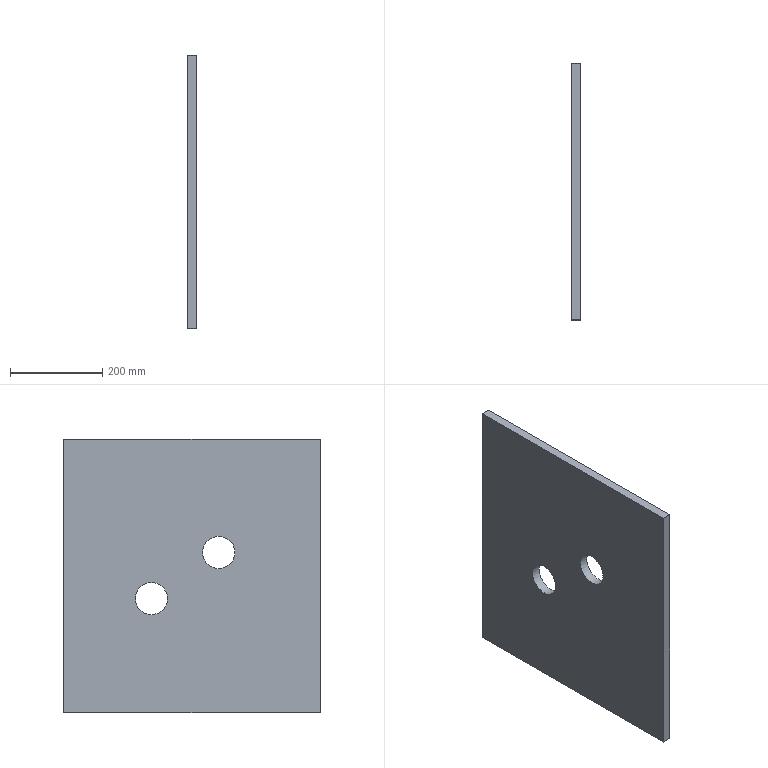Component | NX | BEARING_HOUSING_FIX_PLATE | 1 solid | 8 faces | box 20 x 556 x 594 mm | volume 6451342 mm3 | plane 6 | cylinder 2 | commonest cylinder face diameters 70 x2
STEP:
#1=CARTESIAN_POINT('',(0.,0.,0.));
#2=DIRECTION('',(0.,0.,1.));
#3=DIRECTION('',(1.,0.,0.));
#4=AXIS2_PLACEMENT_3D('',#1,#2,#3);
#5=CARTESIAN_POINT('',(1436.754,3.5,717.5));
#6=VERTEX_POINT('',#5);
#7=CARTESIAN_POINT('',(1436.754,3.5,123.5));
#8=VERTEX_POINT('',#7);
#9=CARTESIAN_POINT('',(1436.754,3.5,717.5));
#10=DIRECTION('',(0.,0.,-1.));
#11=VECTOR('',#10,1.);
#12=LINE('',#9,#11);
#13=CARTESIAN_POINT('',(1456.754,3.5,717.5));
#14=DIRECTION('',(0.,1.,0.));
#15=DIRECTION('',(0.,0.,1.));
#16=AXIS2_PLACEMENT_3D('',#13,#14,#15);
#17=PLANE('',#16);
#18=CARTESIAN_POINT('',(0.,-20.));
#19=DIRECTION('',(-1.,0.));
#20=VECTOR('',#19,1.);
#21=LINE('',#18,#20);
#22=(GEOMETRIC_REPRESENTATION_CONTEXT(2)PARAMETRIC_REPRESENTATION_CONTEXT()REPRESENTATION_CONTEXT('',''));
#23=DEFINITIONAL_REPRESENTATION('',(#21),#22);
#24=PCURVE('',#17,#23);
#25=CARTESIAN_POINT('',(1436.754,223.5,471.5));
#26=DIRECTION('',(1.,0.,0.));
#27=DIRECTION('',(0.,0.,-1.));
#28=AXIS2_PLACEMENT_3D('',#25,#26,#27);
#29=PLANE('',#28);
#30=CARTESIAN_POINT('',(-246.,-220.));
#31=DIRECTION('',(1.,0.));
#32=VECTOR('',#31,1.);
#33=LINE('',#30,#32);
#34=(GEOMETRIC_REPRESENTATION_CONTEXT(2)PARAMETRIC_REPRESENTATION_CONTEXT()REPRESENTATION_CONTEXT('',''));
#35=DEFINITIONAL_REPRESENTATION('',(#33),#34);
#36=PCURVE('',#29,#35);
#37=SURFACE_CURVE('',#12,(#24,#36),.PCURVE_S1.);
#38=EDGE_CURVE('',#6,#8,#37,.T.);
#39=ORIENTED_EDGE('',*,*,#38,.T.);
#40=CARTESIAN_POINT('',(1456.754,3.5,123.5));
#41=VERTEX_POINT('',#40);
#42=CARTESIAN_POINT('',(1456.754,3.5,123.5));
#43=DIRECTION('',(-1.,0.,0.));
#44=VECTOR('',#43,1.);
#45=LINE('',#42,#44);
#46=CARTESIAN_POINT('',(-594.,0.));
#47=DIRECTION('',(0.,-1.));
#48=VECTOR('',#47,1.);
#49=LINE('',#46,#48);
#50=(GEOMETRIC_REPRESENTATION_CONTEXT(2)PARAMETRIC_REPRESENTATION_CONTEXT()REPRESENTATION_CONTEXT('',''));
#51=DEFINITIONAL_REPRESENTATION('',(#49),#50);
#52=PCURVE('',#17,#51);
#53=CARTESIAN_POINT('',(1456.754,3.5,123.5));
#54=DIRECTION('',(0.,0.,1.));
#55=DIRECTION('',(1.,0.,0.));
#56=AXIS2_PLACEMENT_3D('',#53,#54,#55);
#57=PLANE('',#56);
#58=CARTESIAN_POINT('',(0.,0.));
#59=DIRECTION('',(-1.,0.));
#60=VECTOR('',#59,1.);
#61=LINE('',#58,#60);
#62=(GEOMETRIC_REPRESENTATION_CONTEXT(2)PARAMETRIC_REPRESENTATION_CONTEXT()REPRESENTATION_CONTEXT('',''));
#63=DEFINITIONAL_REPRESENTATION('',(#61),#62);
#64=PCURVE('',#57,#63);
#65=SURFACE_CURVE('',#45,(#52,#64),.PCURVE_S1.);
#66=EDGE_CURVE('',#41,#8,#65,.T.);
#67=ORIENTED_EDGE('',*,*,#66,.F.);
#68=CARTESIAN_POINT('',(1456.754,3.5,717.5));
#69=VERTEX_POINT('',#68);
#70=CARTESIAN_POINT('',(1456.754,3.5,717.5));
#71=DIRECTION('',(0.,0.,-1.));
#72=VECTOR('',#71,1.);
#73=LINE('',#70,#72);
#74=CARTESIAN_POINT('',(0.,0.));
#75=DIRECTION('',(-1.,0.));
#76=VECTOR('',#75,1.);
#77=LINE('',#74,#76);
#78=(GEOMETRIC_REPRESENTATION_CONTEXT(2)PARAMETRIC_REPRESENTATION_CONTEXT()REPRESENTATION_CONTEXT('',''));
#79=DEFINITIONAL_REPRESENTATION('',(#77),#78);
#80=PCURVE('',#17,#79);
#81=CARTESIAN_POINT('',(1456.754,223.5,471.5));
#82=DIRECTION('',(1.,0.,0.));
#83=DIRECTION('',(0.,0.,-1.));
#84=AXIS2_PLACEMENT_3D('',#81,#82,#83);
#85=PLANE('',#84);
#86=CARTESIAN_POINT('',(-246.,-220.));
#87=DIRECTION('',(1.,0.));
#88=VECTOR('',#87,1.);
#89=LINE('',#86,#88);
#90=(GEOMETRIC_REPRESENTATION_CONTEXT(2)PARAMETRIC_REPRESENTATION_CONTEXT()REPRESENTATION_CONTEXT('',''));
#91=DEFINITIONAL_REPRESENTATION('',(#89),#90);
#92=PCURVE('',#85,#91);
#93=SURFACE_CURVE('',#73,(#80,#92),.PCURVE_S1.);
#94=EDGE_CURVE('',#69,#41,#93,.T.);
#95=ORIENTED_EDGE('',*,*,#94,.F.);
#96=CARTESIAN_POINT('',(1456.754,3.5,717.5));
#97=DIRECTION('',(-1.,0.,0.));
#98=VECTOR('',#97,1.);
#99=LINE('',#96,#98);
#100=CARTESIAN_POINT('',(0.,0.));
#101=DIRECTION('',(0.,-1.));
#102=VECTOR('',#101,1.);
#103=LINE('',#100,#102);
#104=(GEOMETRIC_REPRESENTATION_CONTEXT(2)PARAMETRIC_REPRESENTATION_CONTEXT()REPRESENTATION_CONTEXT('',''));
#105=DEFINITIONAL_REPRESENTATION('',(#103),#104);
#106=PCURVE('',#17,#105);
#107=CARTESIAN_POINT('',(1456.754,559.5,717.5));
#108=DIRECTION('',(0.,0.,-1.));
#109=DIRECTION('',(-1.,0.,0.));
#110=AXIS2_PLACEMENT_3D('',#107,#108,#109);
#111=PLANE('',#110);
#112=CARTESIAN_POINT('',(0.,-556.));
#113=DIRECTION('',(1.,0.));
#114=VECTOR('',#113,1.);
#115=LINE('',#112,#114);
#116=(GEOMETRIC_REPRESENTATION_CONTEXT(2)PARAMETRIC_REPRESENTATION_CONTEXT()REPRESENTATION_CONTEXT('',''));
#117=DEFINITIONAL_REPRESENTATION('',(#115),#116);
#118=PCURVE('',#111,#117);
#119=SURFACE_CURVE('',#99,(#106,#118),.PCURVE_S1.);
#120=EDGE_CURVE('',#69,#6,#119,.T.);
#121=ORIENTED_EDGE('',*,*,#120,.T.);
#122=EDGE_LOOP('',(#39,#67,#95,#121));
#123=FACE_BOUND('',#122,.T.);
#124=ADVANCED_FACE('',(#123),#17,.F.);
#125=CARTESIAN_POINT('',(1436.754,559.5,123.5));
#126=VERTEX_POINT('',#125);
#127=CARTESIAN_POINT('',(1436.754,3.5,123.5));
#128=DIRECTION('',(0.,1.,0.));
#129=VECTOR('',#128,1.);
#130=LINE('',#127,#129);
#131=CARTESIAN_POINT('',(-20.,0.));
#132=DIRECTION('',(0.,1.));
#133=VECTOR('',#132,1.);
#134=LINE('',#131,#133);
#135=(GEOMETRIC_REPRESENTATION_CONTEXT(2)PARAMETRIC_REPRESENTATION_CONTEXT()REPRESENTATION_CONTEXT('',''));
#136=DEFINITIONAL_REPRESENTATION('',(#134),#135);
#137=PCURVE('',#57,#136);
#138=CARTESIAN_POINT('',(348.,-220.));
#139=DIRECTION('',(0.,1.));
#140=VECTOR('',#139,1.);
#141=LINE('',#138,#140);
#142=(GEOMETRIC_REPRESENTATION_CONTEXT(2)PARAMETRIC_REPRESENTATION_CONTEXT()REPRESENTATION_CONTEXT('',''));
#143=DEFINITIONAL_REPRESENTATION('',(#141),#142);
#144=PCURVE('',#29,#143);
#145=SURFACE_CURVE('',#130,(#137,#144),.PCURVE_S1.);
#146=EDGE_CURVE('',#8,#126,#145,.T.);
#147=ORIENTED_EDGE('',*,*,#146,.T.);
#148=CARTESIAN_POINT('',(1456.754,559.5,123.5));
#149=VERTEX_POINT('',#148);
#150=CARTESIAN_POINT('',(1456.754,559.5,123.5));
#151=DIRECTION('',(-1.,0.,0.));
#152=VECTOR('',#151,1.);
#153=LINE('',#150,#152);
#154=CARTESIAN_POINT('',(0.,556.));
#155=DIRECTION('',(-1.,0.));
#156=VECTOR('',#155,1.);
#157=LINE('',#154,#156);
#158=(GEOMETRIC_REPRESENTATION_CONTEXT(2)PARAMETRIC_REPRESENTATION_CONTEXT()REPRESENTATION_CONTEXT('',''));
#159=DEFINITIONAL_REPRESENTATION('',(#157),#158);
#160=PCURVE('',#57,#159);
#161=CARTESIAN_POINT('',(1456.754,559.5,123.5));
#162=DIRECTION('',(0.,-1.,0.));
#163=DIRECTION('',(0.,0.,-1.));
#164=AXIS2_PLACEMENT_3D('',#161,#162,#163);
#165=PLANE('',#164);
#166=CARTESIAN_POINT('',(0.,0.));
#167=DIRECTION('',(0.,-1.));
#168=VECTOR('',#167,1.);
#169=LINE('',#166,#168);
#170=(GEOMETRIC_REPRESENTATION_CONTEXT(2)PARAMETRIC_REPRESENTATION_CONTEXT()REPRESENTATION_CONTEXT('',''));
#171=DEFINITIONAL_REPRESENTATION('',(#169),#170);
#172=PCURVE('',#165,#171);
#173=SURFACE_CURVE('',#153,(#160,#172),.PCURVE_S1.);
#174=EDGE_CURVE('',#149,#126,#173,.T.);
#175=ORIENTED_EDGE('',*,*,#174,.F.);
#176=CARTESIAN_POINT('',(1456.754,3.5,123.5));
#177=DIRECTION('',(0.,1.,0.));
#178=VECTOR('',#177,1.);
#179=LINE('',#176,#178);
#180=CARTESIAN_POINT('',(0.,0.));
#181=DIRECTION('',(0.,1.));
#182=VECTOR('',#181,1.);
#183=LINE('',#180,#182);
#184=(GEOMETRIC_REPRESENTATION_CONTEXT(2)PARAMETRIC_REPRESENTATION_CONTEXT()REPRESENTATION_CONTEXT('',''));
#185=DEFINITIONAL_REPRESENTATION('',(#183),#184);
#186=PCURVE('',#57,#185);
#187=CARTESIAN_POINT('',(348.,-220.));
#188=DIRECTION('',(0.,1.));
#189=VECTOR('',#188,1.);
#190=LINE('',#187,#189);
#191=(GEOMETRIC_REPRESENTATION_CONTEXT(2)PARAMETRIC_REPRESENTATION_CONTEXT()REPRESENTATION_CONTEXT('',''));
#192=DEFINITIONAL_REPRESENTATION('',(#190),#191);
#193=PCURVE('',#85,#192);
#194=SURFACE_CURVE('',#179,(#186,#193),.PCURVE_S1.);
#195=EDGE_CURVE('',#41,#149,#194,.T.);
#196=ORIENTED_EDGE('',*,*,#195,.F.);
#197=ORIENTED_EDGE('',*,*,#66,.T.);
#198=EDGE_LOOP('',(#147,#175,#196,#197));
#199=FACE_BOUND('',#198,.T.);
#200=ADVANCED_FACE('',(#199),#57,.F.);
#201=CARTESIAN_POINT('',(1436.754,559.5,717.5));
#202=VERTEX_POINT('',#201);
#203=CARTESIAN_POINT('',(1436.754,559.5,123.5));
#204=DIRECTION('',(0.,0.,1.));
#205=VECTOR('',#204,1.);
#206=LINE('',#203,#205);
#207=CARTESIAN_POINT('',(0.,-20.));
#208=DIRECTION('',(-1.,0.));
#209=VECTOR('',#208,1.);
#210=LINE('',#207,#209);
#211=(GEOMETRIC_REPRESENTATION_CONTEXT(2)PARAMETRIC_REPRESENTATION_CONTEXT()REPRESENTATION_CONTEXT('',''));
#212=DEFINITIONAL_REPRESENTATION('',(#210),#211);
#213=PCURVE('',#165,#212);
#214=CARTESIAN_POINT('',(348.,336.));
#215=DIRECTION('',(-1.,0.));
#216=VECTOR('',#215,1.);
#217=LINE('',#214,#216);
#218=(GEOMETRIC_REPRESENTATION_CONTEXT(2)PARAMETRIC_REPRESENTATION_CONTEXT()REPRESENTATION_CONTEXT('',''));
#219=DEFINITIONAL_REPRESENTATION('',(#217),#218);
#220=PCURVE('',#29,#219);
#221=SURFACE_CURVE('',#206,(#213,#220),.PCURVE_S1.);
#222=EDGE_CURVE('',#126,#202,#221,.T.);
#223=ORIENTED_EDGE('',*,*,#222,.T.);
#224=CARTESIAN_POINT('',(1456.754,559.5,717.5));
#225=VERTEX_POINT('',#224);
#226=CARTESIAN_POINT('',(1456.754,559.5,717.5));
#227=DIRECTION('',(-1.,0.,0.));
#228=VECTOR('',#227,1.);
#229=LINE('',#226,#228);
#230=CARTESIAN_POINT('',(-594.,0.));
#231=DIRECTION('',(0.,-1.));
#232=VECTOR('',#231,1.);
#233=LINE('',#230,#232);
#234=(GEOMETRIC_REPRESENTATION_CONTEXT(2)PARAMETRIC_REPRESENTATION_CONTEXT()REPRESENTATION_CONTEXT('',''));
#235=DEFINITIONAL_REPRESENTATION('',(#233),#234);
#236=PCURVE('',#165,#235);
#237=CARTESIAN_POINT('',(0.,0.));
#238=DIRECTION('',(1.,0.));
#239=VECTOR('',#238,1.);
#240=LINE('',#237,#239);
#241=(GEOMETRIC_REPRESENTATION_CONTEXT(2)PARAMETRIC_REPRESENTATION_CONTEXT()REPRESENTATION_CONTEXT('',''));
#242=DEFINITIONAL_REPRESENTATION('',(#240),#241);
#243=PCURVE('',#111,#242);
#244=SURFACE_CURVE('',#229,(#236,#243),.PCURVE_S1.);
#245=EDGE_CURVE('',#225,#202,#244,.T.);
#246=ORIENTED_EDGE('',*,*,#245,.F.);
#247=CARTESIAN_POINT('',(1456.754,559.5,123.5));
#248=DIRECTION('',(0.,0.,1.));
#249=VECTOR('',#248,1.);
#250=LINE('',#247,#249);
#251=CARTESIAN_POINT('',(0.,0.));
#252=DIRECTION('',(-1.,0.));
#253=VECTOR('',#252,1.);
#254=LINE('',#251,#253);
#255=(GEOMETRIC_REPRESENTATION_CONTEXT(2)PARAMETRIC_REPRESENTATION_CONTEXT()REPRESENTATION_CONTEXT('',''));
#256=DEFINITIONAL_REPRESENTATION('',(#254),#255);
#257=PCURVE('',#165,#256);
#258=CARTESIAN_POINT('',(348.,336.));
#259=DIRECTION('',(-1.,0.));
#260=VECTOR('',#259,1.);
#261=LINE('',#258,#260);
#262=(GEOMETRIC_REPRESENTATION_CONTEXT(2)PARAMETRIC_REPRESENTATION_CONTEXT()REPRESENTATION_CONTEXT('',''));
#263=DEFINITIONAL_REPRESENTATION('',(#261),#262);
#264=PCURVE('',#85,#263);
#265=SURFACE_CURVE('',#250,(#257,#264),.PCURVE_S1.);
#266=EDGE_CURVE('',#149,#225,#265,.T.);
#267=ORIENTED_EDGE('',*,*,#266,.F.);
#268=ORIENTED_EDGE('',*,*,#174,.T.);
#269=EDGE_LOOP('',(#223,#246,#267,#268));
#270=FACE_BOUND('',#269,.T.);
#271=ADVANCED_FACE('',(#270),#165,.F.);
#272=CARTESIAN_POINT('',(1456.754,258.5,471.5));
#273=VERTEX_POINT('',#272);
#274=CARTESIAN_POINT('',(1456.754,223.5,471.5));
#275=DIRECTION('',(1.,0.,0.));
#276=DIRECTION('',(0.,1.,0.));
#277=AXIS2_PLACEMENT_3D('',#274,#275,#276);
#278=CIRCLE('',#277,35.);
#279=CARTESIAN_POINT('',(1456.754,223.5,471.5));
#280=DIRECTION('',(-1.,0.,0.));
#281=DIRECTION('',(0.,0.,1.));
#282=AXIS2_PLACEMENT_3D('',#279,#280,#281);
#283=CYLINDRICAL_SURFACE('',#282,35.);
#284=CARTESIAN_POINT('',(7.854,0.));
#285=DIRECTION('',(-1.,0.));
#286=VECTOR('',#285,1.);
#287=LINE('',#284,#286);
#288=(GEOMETRIC_REPRESENTATION_CONTEXT(2)PARAMETRIC_REPRESENTATION_CONTEXT()REPRESENTATION_CONTEXT('',''));
#289=DEFINITIONAL_REPRESENTATION('',(#287),#288);
#290=PCURVE('',#283,#289);
#291=CARTESIAN_POINT('',(0.,0.));
#292=DIRECTION('',(0.,1.));
#293=AXIS2_PLACEMENT_2D('',#291,#292);
#294=CIRCLE('',#293,35.);
#295=(GEOMETRIC_REPRESENTATION_CONTEXT(2)PARAMETRIC_REPRESENTATION_CONTEXT()REPRESENTATION_CONTEXT('',''));
#296=DEFINITIONAL_REPRESENTATION('',(#294),#295);
#297=PCURVE('',#85,#296);
#298=SURFACE_CURVE('',#278,(#290,#297),.PCURVE_S1.);
#299=EDGE_CURVE('',#273,#273,#298,.T.);
#300=ORIENTED_EDGE('',*,*,#299,.F.);
#301=CARTESIAN_POINT('',(1436.754,258.5,471.5));
#302=VERTEX_POINT('',#301);
#303=CARTESIAN_POINT('',(1456.754,258.5,471.5));
#304=CARTESIAN_POINT('',(1436.754,258.5,471.5));
#305=B_SPLINE_CURVE_WITH_KNOTS('',1,(#303,#304),.UNSPECIFIED.,.F.,.F.,(2,2),(0.,20.),.PIECEWISE_BEZIER_KNOTS.);
#306=CARTESIAN_POINT('',(7.854,0.));
#307=DIRECTION('',(0.,1.));
#308=VECTOR('',#307,1.);
#309=LINE('',#306,#308);
#310=(GEOMETRIC_REPRESENTATION_CONTEXT(2)PARAMETRIC_REPRESENTATION_CONTEXT()REPRESENTATION_CONTEXT('',''));
#311=DEFINITIONAL_REPRESENTATION('',(#309),#310);
#312=PCURVE('',#283,#311);
#313=CARTESIAN_POINT('',(1.571,0.));
#314=DIRECTION('',(0.,1.));
#315=VECTOR('',#314,1.);
#316=LINE('',#313,#315);
#317=(GEOMETRIC_REPRESENTATION_CONTEXT(2)PARAMETRIC_REPRESENTATION_CONTEXT()REPRESENTATION_CONTEXT('',''));
#318=DEFINITIONAL_REPRESENTATION('',(#316),#317);
#319=PCURVE('',#283,#318);
#320=SEAM_CURVE('',#305,(#312,#319),.PCURVE_S1.);
#321=EDGE_CURVE('',#273,#302,#320,.T.);
#322=ORIENTED_EDGE('',*,*,#321,.T.);
#323=CARTESIAN_POINT('',(1436.754,223.5,471.5));
#324=DIRECTION('',(1.,0.,0.));
#325=DIRECTION('',(0.,1.,0.));
#326=AXIS2_PLACEMENT_3D('',#323,#324,#325);
#327=CIRCLE('',#326,35.);
#328=CARTESIAN_POINT('',(7.854,20.));
#329=DIRECTION('',(-1.,0.));
#330=VECTOR('',#329,1.);
#331=LINE('',#328,#330);
#332=(GEOMETRIC_REPRESENTATION_CONTEXT(2)PARAMETRIC_REPRESENTATION_CONTEXT()REPRESENTATION_CONTEXT('',''));
#333=DEFINITIONAL_REPRESENTATION('',(#331),#332);
#334=PCURVE('',#283,#333);
#335=CARTESIAN_POINT('',(0.,0.));
#336=DIRECTION('',(0.,1.));
#337=AXIS2_PLACEMENT_2D('',#335,#336);
#338=CIRCLE('',#337,35.);
#339=(GEOMETRIC_REPRESENTATION_CONTEXT(2)PARAMETRIC_REPRESENTATION_CONTEXT()REPRESENTATION_CONTEXT('',''));
#340=DEFINITIONAL_REPRESENTATION('',(#338),#339);
#341=PCURVE('',#29,#340);
#342=SURFACE_CURVE('',#327,(#334,#341),.PCURVE_S1.);
#343=EDGE_CURVE('',#302,#302,#342,.T.);
#344=ORIENTED_EDGE('',*,*,#343,.T.);
#345=ORIENTED_EDGE('',*,*,#321,.F.);
#346=EDGE_LOOP('',(#300,#322,#344,#345));
#347=FACE_BOUND('',#346,.F.);
#348=ADVANCED_FACE('',(#347),#283,.F.);
#349=CARTESIAN_POINT('',(1436.754,559.5,717.5));
#350=DIRECTION('',(0.,-1.,0.));
#351=VECTOR('',#350,1.);
#352=LINE('',#349,#351);
#353=CARTESIAN_POINT('',(20.,0.));
#354=DIRECTION('',(0.,-1.));
#355=VECTOR('',#354,1.);
#356=LINE('',#353,#355);
#357=(GEOMETRIC_REPRESENTATION_CONTEXT(2)PARAMETRIC_REPRESENTATION_CONTEXT()REPRESENTATION_CONTEXT('',''));
#358=DEFINITIONAL_REPRESENTATION('',(#356),#357);
#359=PCURVE('',#111,#358);
#360=CARTESIAN_POINT('',(-246.,336.));
#361=DIRECTION('',(0.,-1.));
#362=VECTOR('',#361,1.);
#363=LINE('',#360,#362);
#364=(GEOMETRIC_REPRESENTATION_CONTEXT(2)PARAMETRIC_REPRESENTATION_CONTEXT()REPRESENTATION_CONTEXT('',''));
#365=DEFINITIONAL_REPRESENTATION('',(#363),#364);
#366=PCURVE('',#29,#365);
#367=SURFACE_CURVE('',#352,(#359,#366),.PCURVE_S1.);
#368=EDGE_CURVE('',#202,#6,#367,.T.);
#369=ORIENTED_EDGE('',*,*,#368,.T.);
#370=ORIENTED_EDGE('',*,*,#120,.F.);
#371=CARTESIAN_POINT('',(1456.754,559.5,717.5));
#372=DIRECTION('',(0.,-1.,0.));
#373=VECTOR('',#372,1.);
#374=LINE('',#371,#373);
#375=CARTESIAN_POINT('',(0.,0.));
#376=DIRECTION('',(0.,-1.));
#377=VECTOR('',#376,1.);
#378=LINE('',#375,#377);
#379=(GEOMETRIC_REPRESENTATION_CONTEXT(2)PARAMETRIC_REPRESENTATION_CONTEXT()REPRESENTATION_CONTEXT('',''));
#380=DEFINITIONAL_REPRESENTATION('',(#378),#379);
#381=PCURVE('',#111,#380);
#382=CARTESIAN_POINT('',(-246.,336.));
#383=DIRECTION('',(0.,-1.));
#384=VECTOR('',#383,1.);
#385=LINE('',#382,#384);
#386=(GEOMETRIC_REPRESENTATION_CONTEXT(2)PARAMETRIC_REPRESENTATION_CONTEXT()REPRESENTATION_CONTEXT('',''));
#387=DEFINITIONAL_REPRESENTATION('',(#385),#386);
#388=PCURVE('',#85,#387);
#389=SURFACE_CURVE('',#374,(#381,#388),.PCURVE_S1.);
#390=EDGE_CURVE('',#225,#69,#389,.T.);
#391=ORIENTED_EDGE('',*,*,#390,.F.);
#392=ORIENTED_EDGE('',*,*,#245,.T.);
#393=EDGE_LOOP('',(#369,#370,#391,#392));
#394=FACE_BOUND('',#393,.T.);
#395=ADVANCED_FACE('',(#394),#111,.F.);
#396=CARTESIAN_POINT('',(1456.754,404.5,371.5));
#397=VERTEX_POINT('',#396);
#398=CARTESIAN_POINT('',(1456.754,369.5,371.5));
#399=DIRECTION('',(1.,0.,0.));
#400=DIRECTION('',(0.,1.,0.));
#401=AXIS2_PLACEMENT_3D('',#398,#399,#400);
#402=CIRCLE('',#401,35.);
#403=CARTESIAN_POINT('',(1456.754,369.5,371.5));
#404=DIRECTION('',(-1.,0.,0.));
#405=DIRECTION('',(0.,0.,1.));
#406=AXIS2_PLACEMENT_3D('',#403,#404,#405);
#407=CYLINDRICAL_SURFACE('',#406,35.);
#408=CARTESIAN_POINT('',(7.854,0.));
#409=DIRECTION('',(-1.,0.));
#410=VECTOR('',#409,1.);
#411=LINE('',#408,#410);
#412=(GEOMETRIC_REPRESENTATION_CONTEXT(2)PARAMETRIC_REPRESENTATION_CONTEXT()REPRESENTATION_CONTEXT('',''));
#413=DEFINITIONAL_REPRESENTATION('',(#411),#412);
#414=PCURVE('',#407,#413);
#415=CARTESIAN_POINT('',(100.,146.));
#416=DIRECTION('',(0.,1.));
#417=AXIS2_PLACEMENT_2D('',#415,#416);
#418=CIRCLE('',#417,35.);
#419=(GEOMETRIC_REPRESENTATION_CONTEXT(2)PARAMETRIC_REPRESENTATION_CONTEXT()REPRESENTATION_CONTEXT('',''));
#420=DEFINITIONAL_REPRESENTATION('',(#418),#419);
#421=PCURVE('',#85,#420);
#422=SURFACE_CURVE('',#402,(#414,#421),.PCURVE_S1.);
#423=EDGE_CURVE('',#397,#397,#422,.T.);
#424=ORIENTED_EDGE('',*,*,#423,.F.);
#425=CARTESIAN_POINT('',(1436.754,404.5,371.5));
#426=VERTEX_POINT('',#425);
#427=CARTESIAN_POINT('',(1456.754,404.5,371.5));
#428=CARTESIAN_POINT('',(1436.754,404.5,371.5));
#429=B_SPLINE_CURVE_WITH_KNOTS('',1,(#427,#428),.UNSPECIFIED.,.F.,.F.,(2,2),(0.,20.),.PIECEWISE_BEZIER_KNOTS.);
#430=CARTESIAN_POINT('',(7.854,0.));
#431=DIRECTION('',(0.,1.));
#432=VECTOR('',#431,1.);
#433=LINE('',#430,#432);
#434=(GEOMETRIC_REPRESENTATION_CONTEXT(2)PARAMETRIC_REPRESENTATION_CONTEXT()REPRESENTATION_CONTEXT('',''));
#435=DEFINITIONAL_REPRESENTATION('',(#433),#434);
#436=PCURVE('',#407,#435);
#437=CARTESIAN_POINT('',(1.571,0.));
#438=DIRECTION('',(0.,1.));
#439=VECTOR('',#438,1.);
#440=LINE('',#437,#439);
#441=(GEOMETRIC_REPRESENTATION_CONTEXT(2)PARAMETRIC_REPRESENTATION_CONTEXT()REPRESENTATION_CONTEXT('',''));
#442=DEFINITIONAL_REPRESENTATION('',(#440),#441);
#443=PCURVE('',#407,#442);
#444=SEAM_CURVE('',#429,(#436,#443),.PCURVE_S1.);
#445=EDGE_CURVE('',#397,#426,#444,.T.);
#446=ORIENTED_EDGE('',*,*,#445,.T.);
#447=CARTESIAN_POINT('',(1436.754,369.5,371.5));
#448=DIRECTION('',(1.,0.,0.));
#449=DIRECTION('',(0.,1.,0.));
#450=AXIS2_PLACEMENT_3D('',#447,#448,#449);
#451=CIRCLE('',#450,35.);
#452=CARTESIAN_POINT('',(7.854,20.));
#453=DIRECTION('',(-1.,0.));
#454=VECTOR('',#453,1.);
#455=LINE('',#452,#454);
#456=(GEOMETRIC_REPRESENTATION_CONTEXT(2)PARAMETRIC_REPRESENTATION_CONTEXT()REPRESENTATION_CONTEXT('',''));
#457=DEFINITIONAL_REPRESENTATION('',(#455),#456);
#458=PCURVE('',#407,#457);
#459=CARTESIAN_POINT('',(100.,146.));
#460=DIRECTION('',(0.,1.));
#461=AXIS2_PLACEMENT_2D('',#459,#460);
#462=CIRCLE('',#461,35.);
#463=(GEOMETRIC_REPRESENTATION_CONTEXT(2)PARAMETRIC_REPRESENTATION_CONTEXT()REPRESENTATION_CONTEXT('',''));
#464=DEFINITIONAL_REPRESENTATION('',(#462),#463);
#465=PCURVE('',#29,#464);
#466=SURFACE_CURVE('',#451,(#458,#465),.PCURVE_S1.);
#467=EDGE_CURVE('',#426,#426,#466,.T.);
#468=ORIENTED_EDGE('',*,*,#467,.T.);
#469=ORIENTED_EDGE('',*,*,#445,.F.);
#470=EDGE_LOOP('',(#424,#446,#468,#469));
#471=FACE_BOUND('',#470,.F.);
#472=ADVANCED_FACE('',(#471),#407,.F.);
#473=ORIENTED_EDGE('',*,*,#94,.T.);
#474=ORIENTED_EDGE('',*,*,#195,.T.);
#475=ORIENTED_EDGE('',*,*,#266,.T.);
#476=ORIENTED_EDGE('',*,*,#390,.T.);
#477=EDGE_LOOP('',(#473,#474,#475,#476));
#478=FACE_BOUND('',#477,.T.);
#479=ORIENTED_EDGE('',*,*,#299,.F.);
#480=EDGE_LOOP('',(#479));
#481=FACE_BOUND('',#480,.T.);
#482=ORIENTED_EDGE('',*,*,#423,.F.);
#483=EDGE_LOOP('',(#482));
#484=FACE_BOUND('',#483,.T.);
#485=ADVANCED_FACE('',(#478,#481,#484),#85,.T.);
#486=ORIENTED_EDGE('',*,*,#38,.F.);
#487=ORIENTED_EDGE('',*,*,#368,.F.);
#488=ORIENTED_EDGE('',*,*,#222,.F.);
#489=ORIENTED_EDGE('',*,*,#146,.F.);
#490=EDGE_LOOP('',(#486,#487,#488,#489));
#491=FACE_BOUND('',#490,.T.);
#492=ORIENTED_EDGE('',*,*,#343,.T.);
#493=EDGE_LOOP('',(#492));
#494=FACE_BOUND('',#493,.T.);
#495=ORIENTED_EDGE('',*,*,#467,.T.);
#496=EDGE_LOOP('',(#495));
#497=FACE_BOUND('',#496,.T.);
#498=ADVANCED_FACE('',(#491,#494,#497),#29,.F.);
#499=CLOSED_SHELL('',(#124,#200,#271,#348,#395,#472,#485,#498));
#500=MANIFOLD_SOLID_BREP('',#499);
#501=(LENGTH_UNIT()NAMED_UNIT(*)SI_UNIT(.MILLI.,.METRE.));
#502=UNCERTAINTY_MEASURE_WITH_UNIT(LENGTH_MEASURE(0.000002),#501,'','');
#503=(NAMED_UNIT(*)PLANE_ANGLE_UNIT()SI_UNIT($,.RADIAN.));
#504=(NAMED_UNIT(*)SI_UNIT($,.STERADIAN.)SOLID_ANGLE_UNIT());
#505=(GEOMETRIC_REPRESENTATION_CONTEXT(3)GLOBAL_UNCERTAINTY_ASSIGNED_CONTEXT((#502))GLOBAL_UNIT_ASSIGNED_CONTEXT((#501,#503,#504))REPRESENTATION_CONTEXT('',''));
#506=ADVANCED_BREP_SHAPE_REPRESENTATION('',(#4,#500),#505);